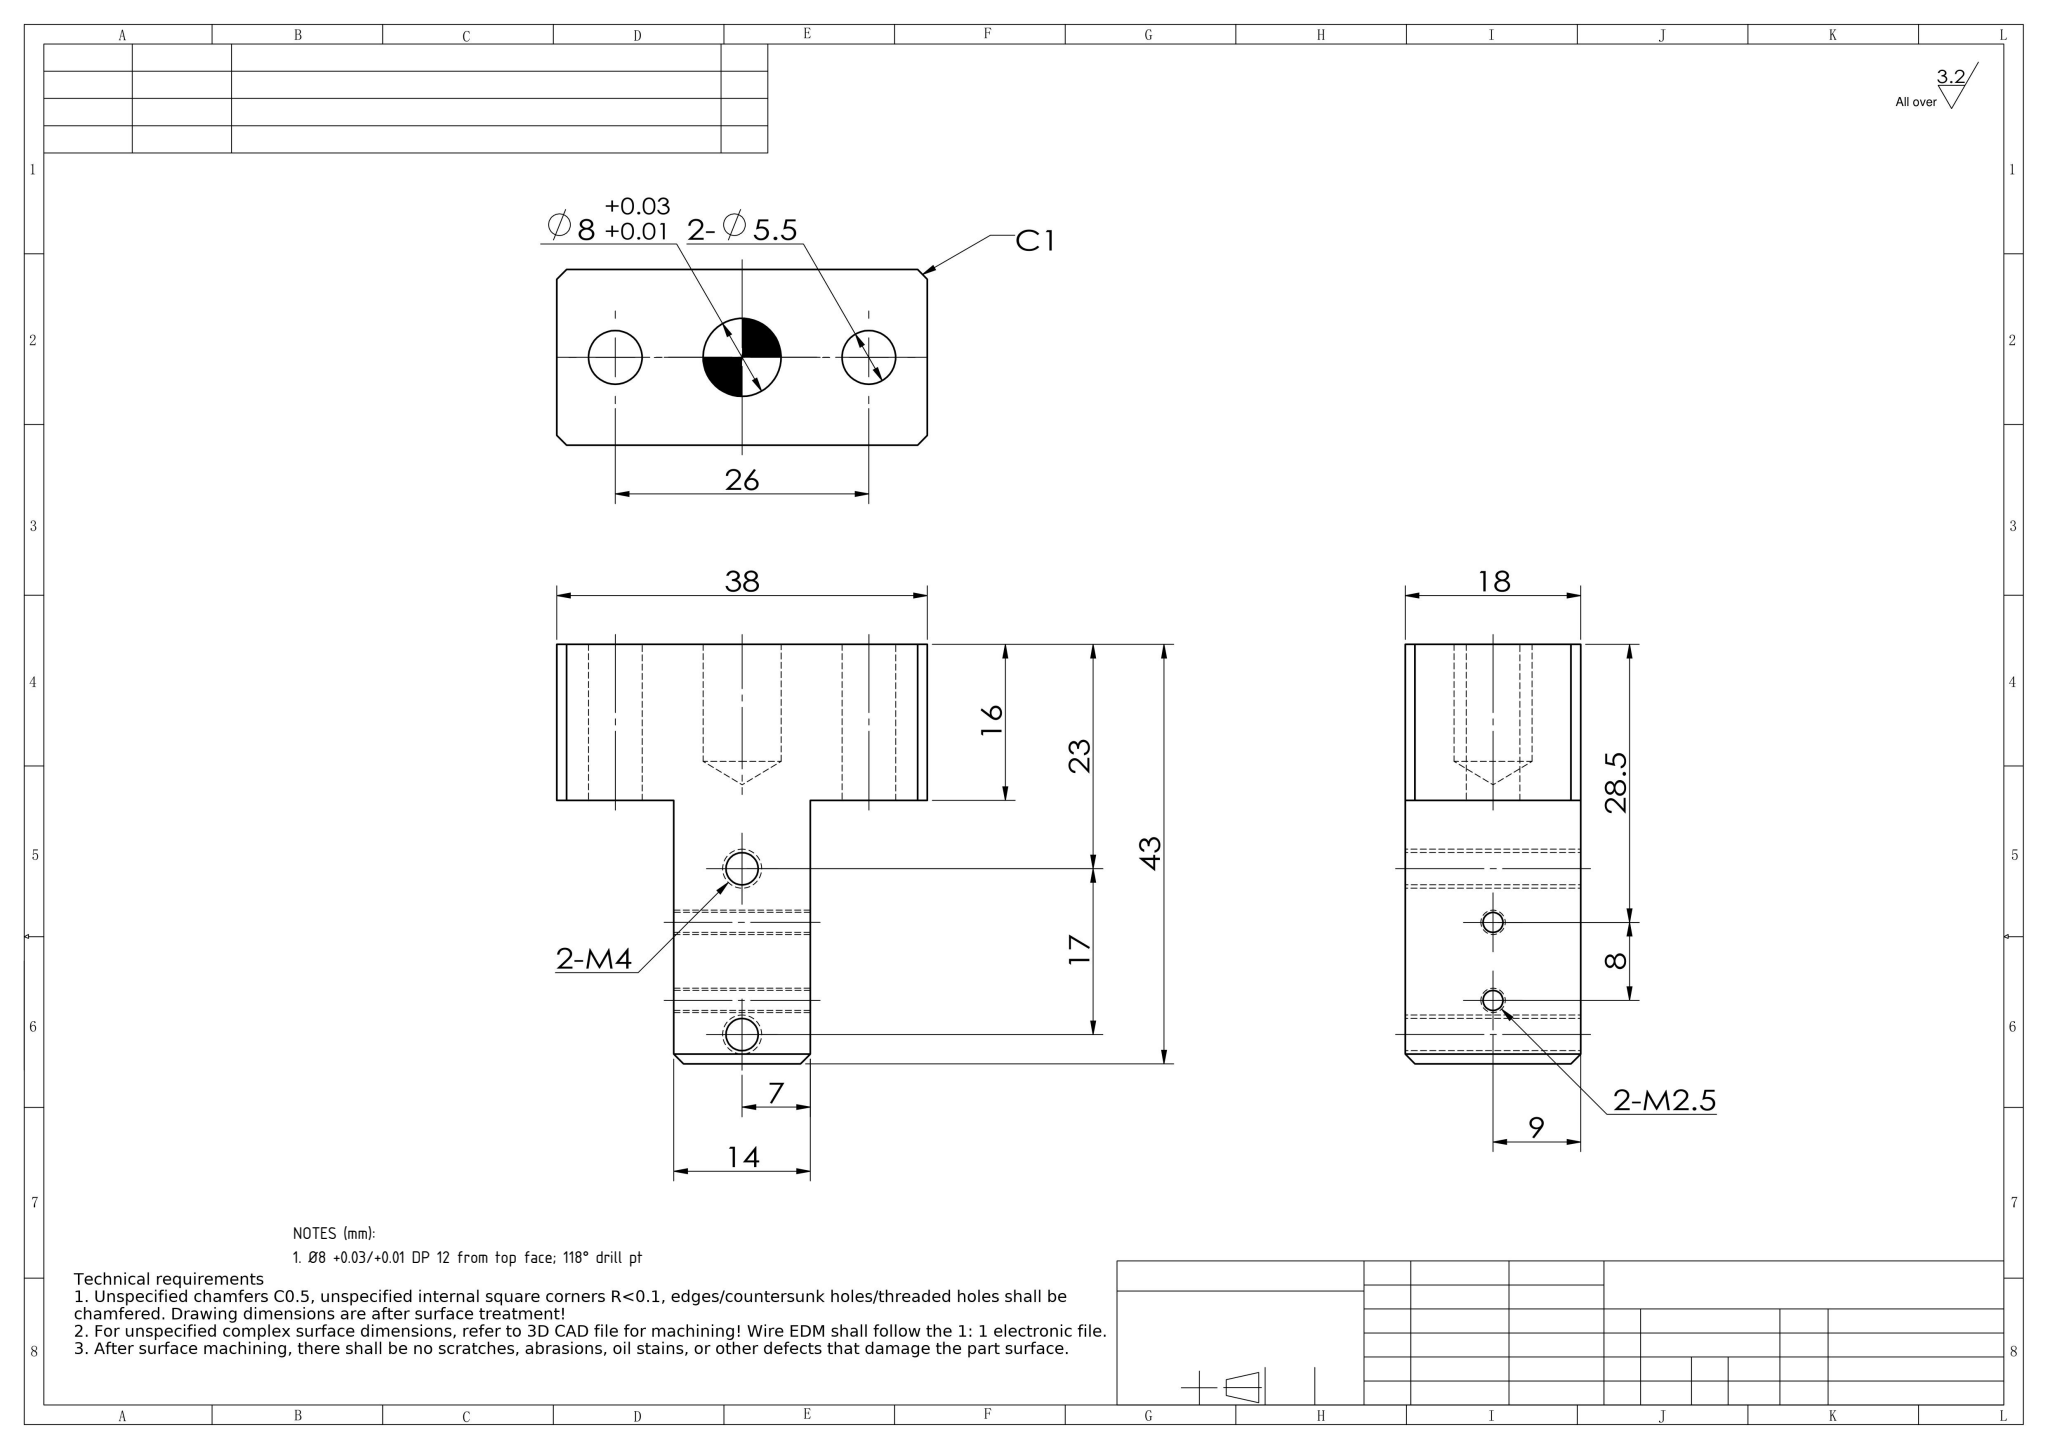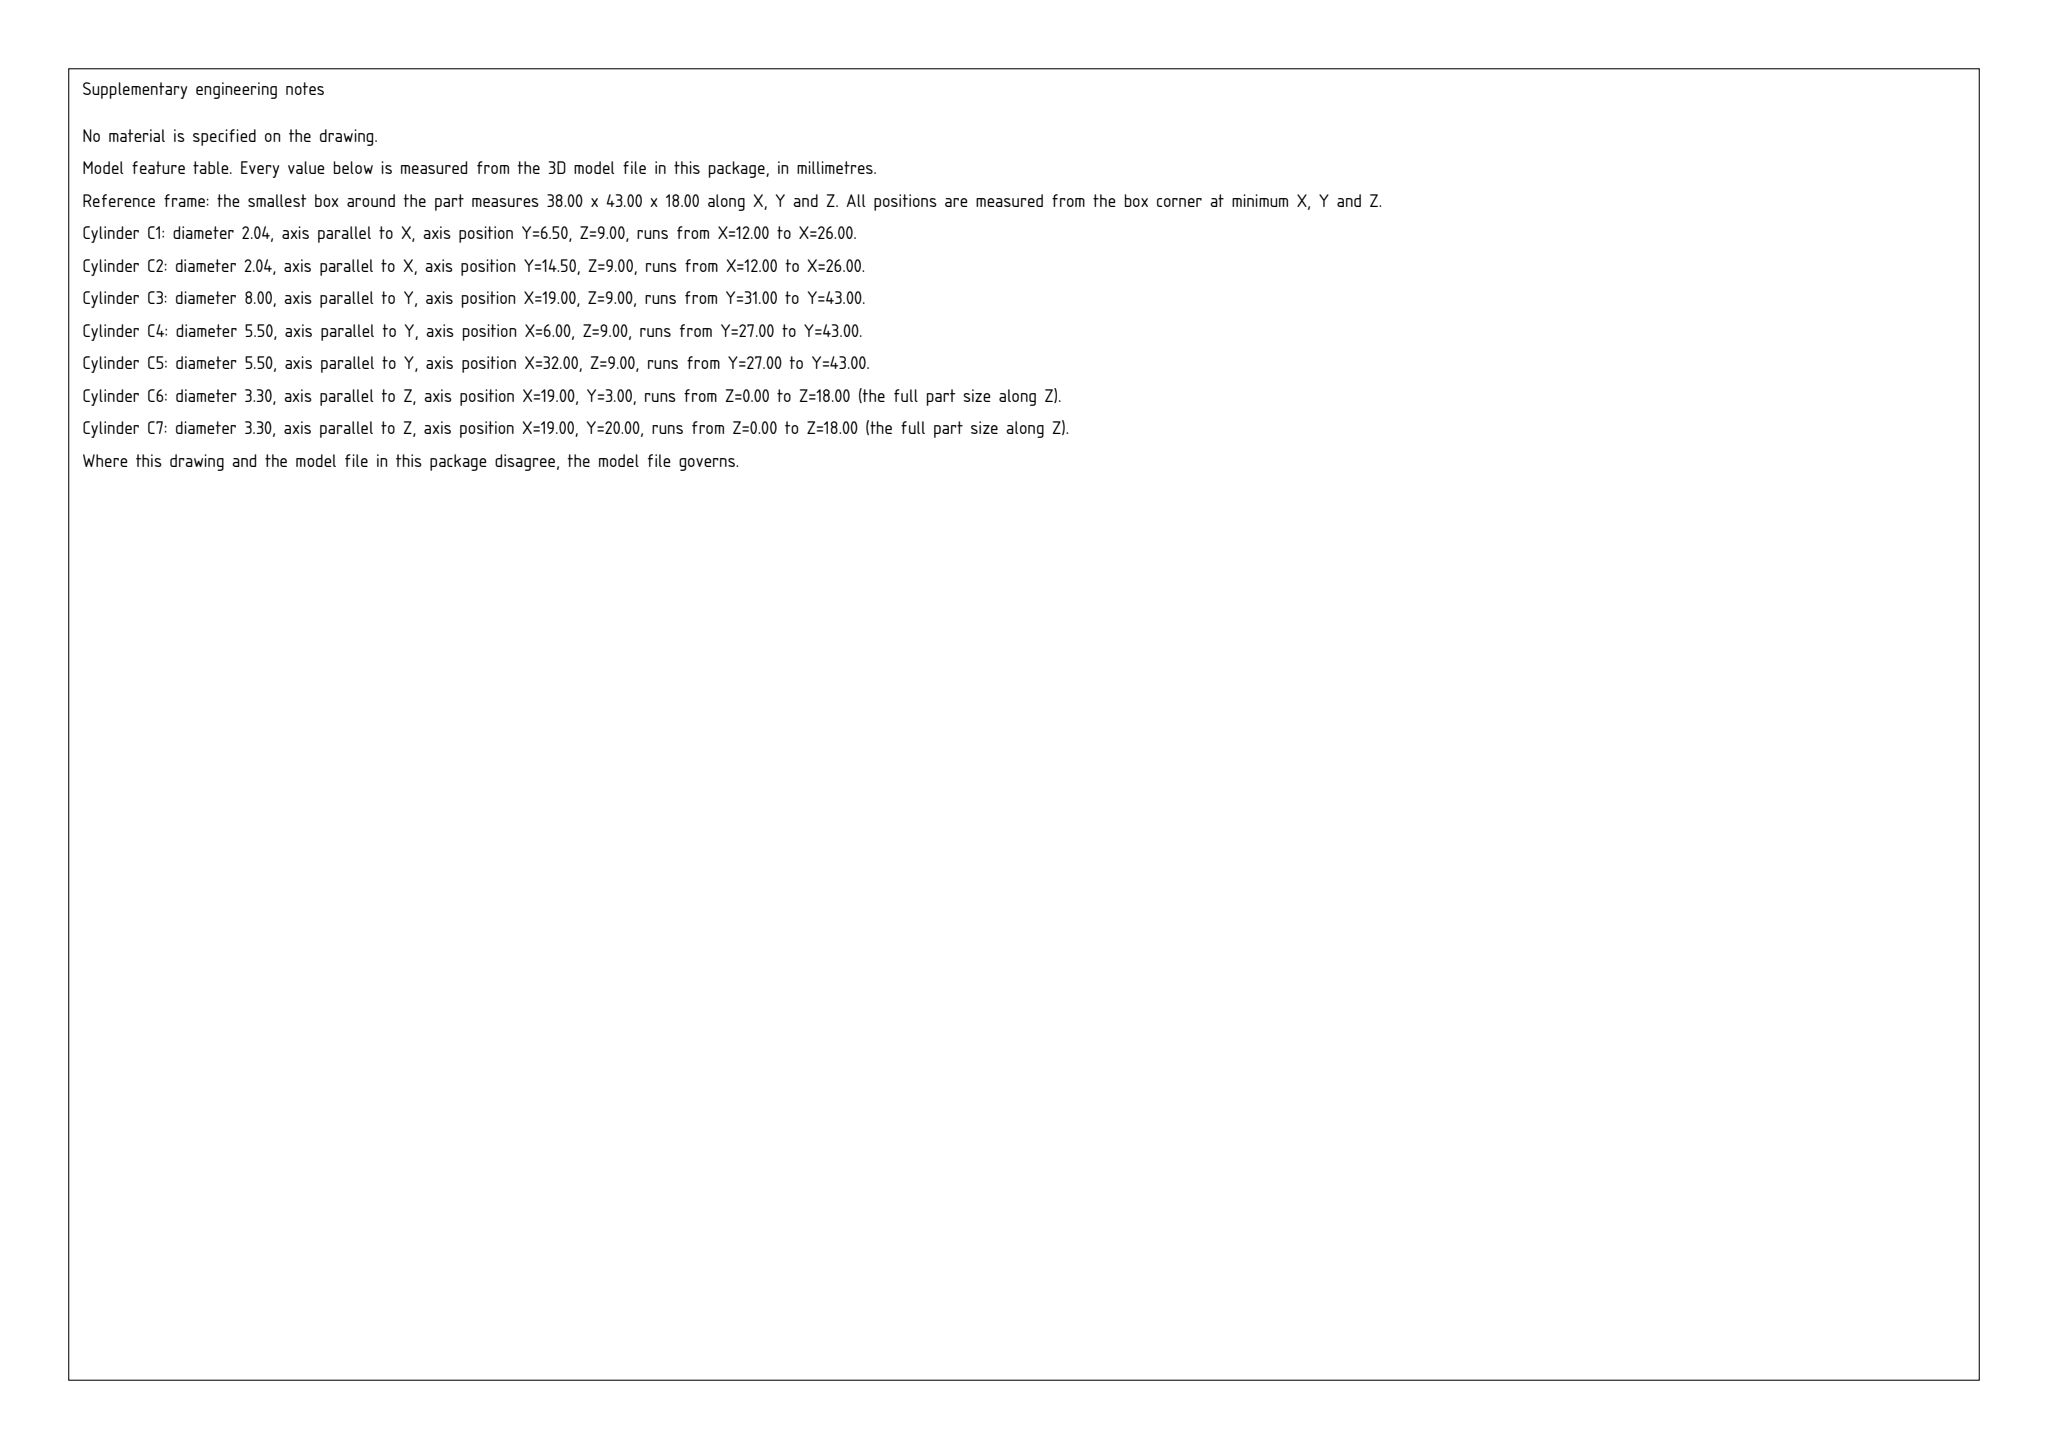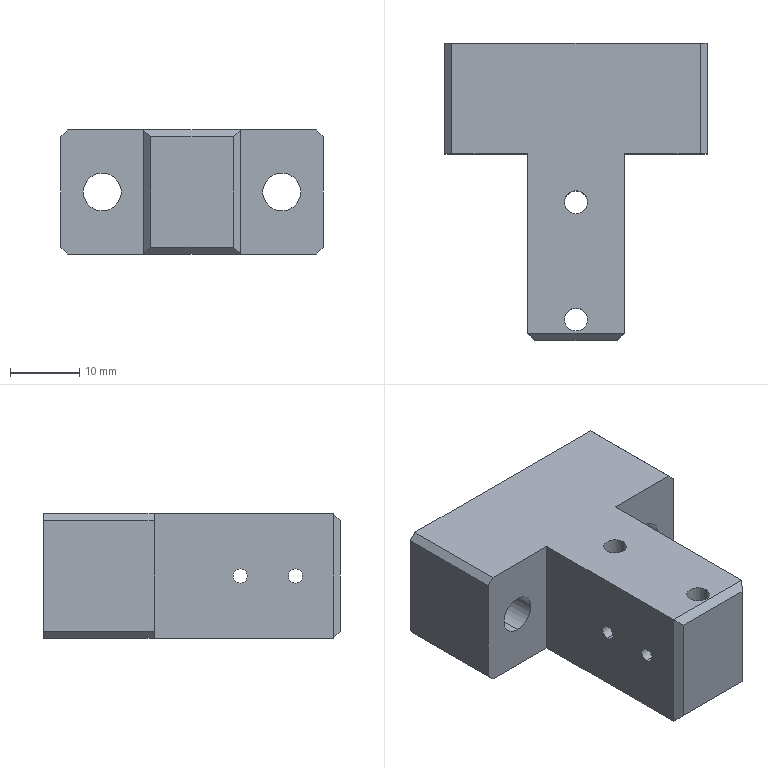Part | SolidWorks | mm | 1 solid | 34 faces | box 38 x 43 x 18 mm | volume 15881 mm3 | plane 18 | cylinder 14 | cone 2 | commonest cylinder face diameters 2.05 x4 3.3 x4 5.5 x4 8 x2
Drawing notes:
Ø8 +0.03/+0.01 DP 12 from top face; 118° drill pt | from the solid: cyl dia 8.0 axis y at (x19,z9) len 12 from y=43 top face; cone 118° ref dia 8
build123d program:
from build123d import *

# Parameters (mm, degrees)
BOSS_EXTRUDE1_DEPTH            = 9
F_5_5_5_5_DIAMETER_HOLE1_D     = 5.5
SIZE_MM_DOWEL_PIN_HOLE_1_D     = 8
SIZE_MM_DOWEL_PIN_HOLE_1_DEPTH = 12
SIZE_MM_DOWEL_PIN_HOLE_1_TIP   = 2.403
M4_TAPPED_HOLE1_D              = 3.3
M2_5_TAPPED_HOLE2_D            = 2.05
CHAMFER1_SIZE                  = 1


with BuildPart() as part:
    # Sketch1 → Boss-Extrude1 (new, symmetric)
    with BuildSketch(Plane.XY):
        Polygon((-19, 5.5), (-7, 5.5), (-7, -21.5), (7, -21.5), (7, 5.5), (19, 5.5), (19, 21.5), (-19, 21.5), align=None)
    extrude(amount=BOSS_EXTRUDE1_DEPTH, both=True)

    # 5.5 _5.5_ Diameter Hole1 (through all)
    with Locations(Plane(origin=(0, 5.5, 0), x_dir=(-1, 0, 0), z_dir=(0, -1, 0))):
        with Locations((-13, 0), (13, 0)):
            Hole(F_5_5_5_5_DIAMETER_HOLE1_D / 2)

    # Size mm Dowel Pin Hole 1
    with Locations(Plane(origin=(0, 21.5, 0), x_dir=(1, 0, 0), z_dir=(0, 1, 0))):
        with Locations((0, 0)):
            Hole(SIZE_MM_DOWEL_PIN_HOLE_1_D / 2, depth=SIZE_MM_DOWEL_PIN_HOLE_1_DEPTH)
            with Locations((0, 0, -(SIZE_MM_DOWEL_PIN_HOLE_1_DEPTH + SIZE_MM_DOWEL_PIN_HOLE_1_TIP / 2))):  # 118° drill point
                Cone(0, SIZE_MM_DOWEL_PIN_HOLE_1_D / 2, SIZE_MM_DOWEL_PIN_HOLE_1_TIP, mode=Mode.SUBTRACT)

    # M4 Tapped Hole1 (through all)
    with Locations(Plane(origin=(0, 0, -9), x_dir=(-1, 0, 0), z_dir=(0, 0, -1))):
        with Locations((0, -18.5), (0, -1.5)):
            Hole(M4_TAPPED_HOLE1_D / 2)

    # M2.5 Tapped Hole2 (through all)
    with Locations(Plane.ZY.offset(7)):
        with Locations((0, -15), (0, -7)):
            Hole(M2_5_TAPPED_HOLE2_D / 2)

    # Chamfer1
    chamfer1_edges = [part.edges().sort_by_distance(p)[0] for p in [
        (-19, 13.5, -9),
        (0, -21.5, 9),
        (7, -21.5, 0),
        (-7, -21.5, 0),
        (19, 13.5, 9),
        (-19, 13.5, 9),
        (19, 13.5, -9),
        (0, -21.5, -9),
    ]]
    chamfer(chamfer1_edges, length=CHAMFER1_SIZE)


solid = part.part